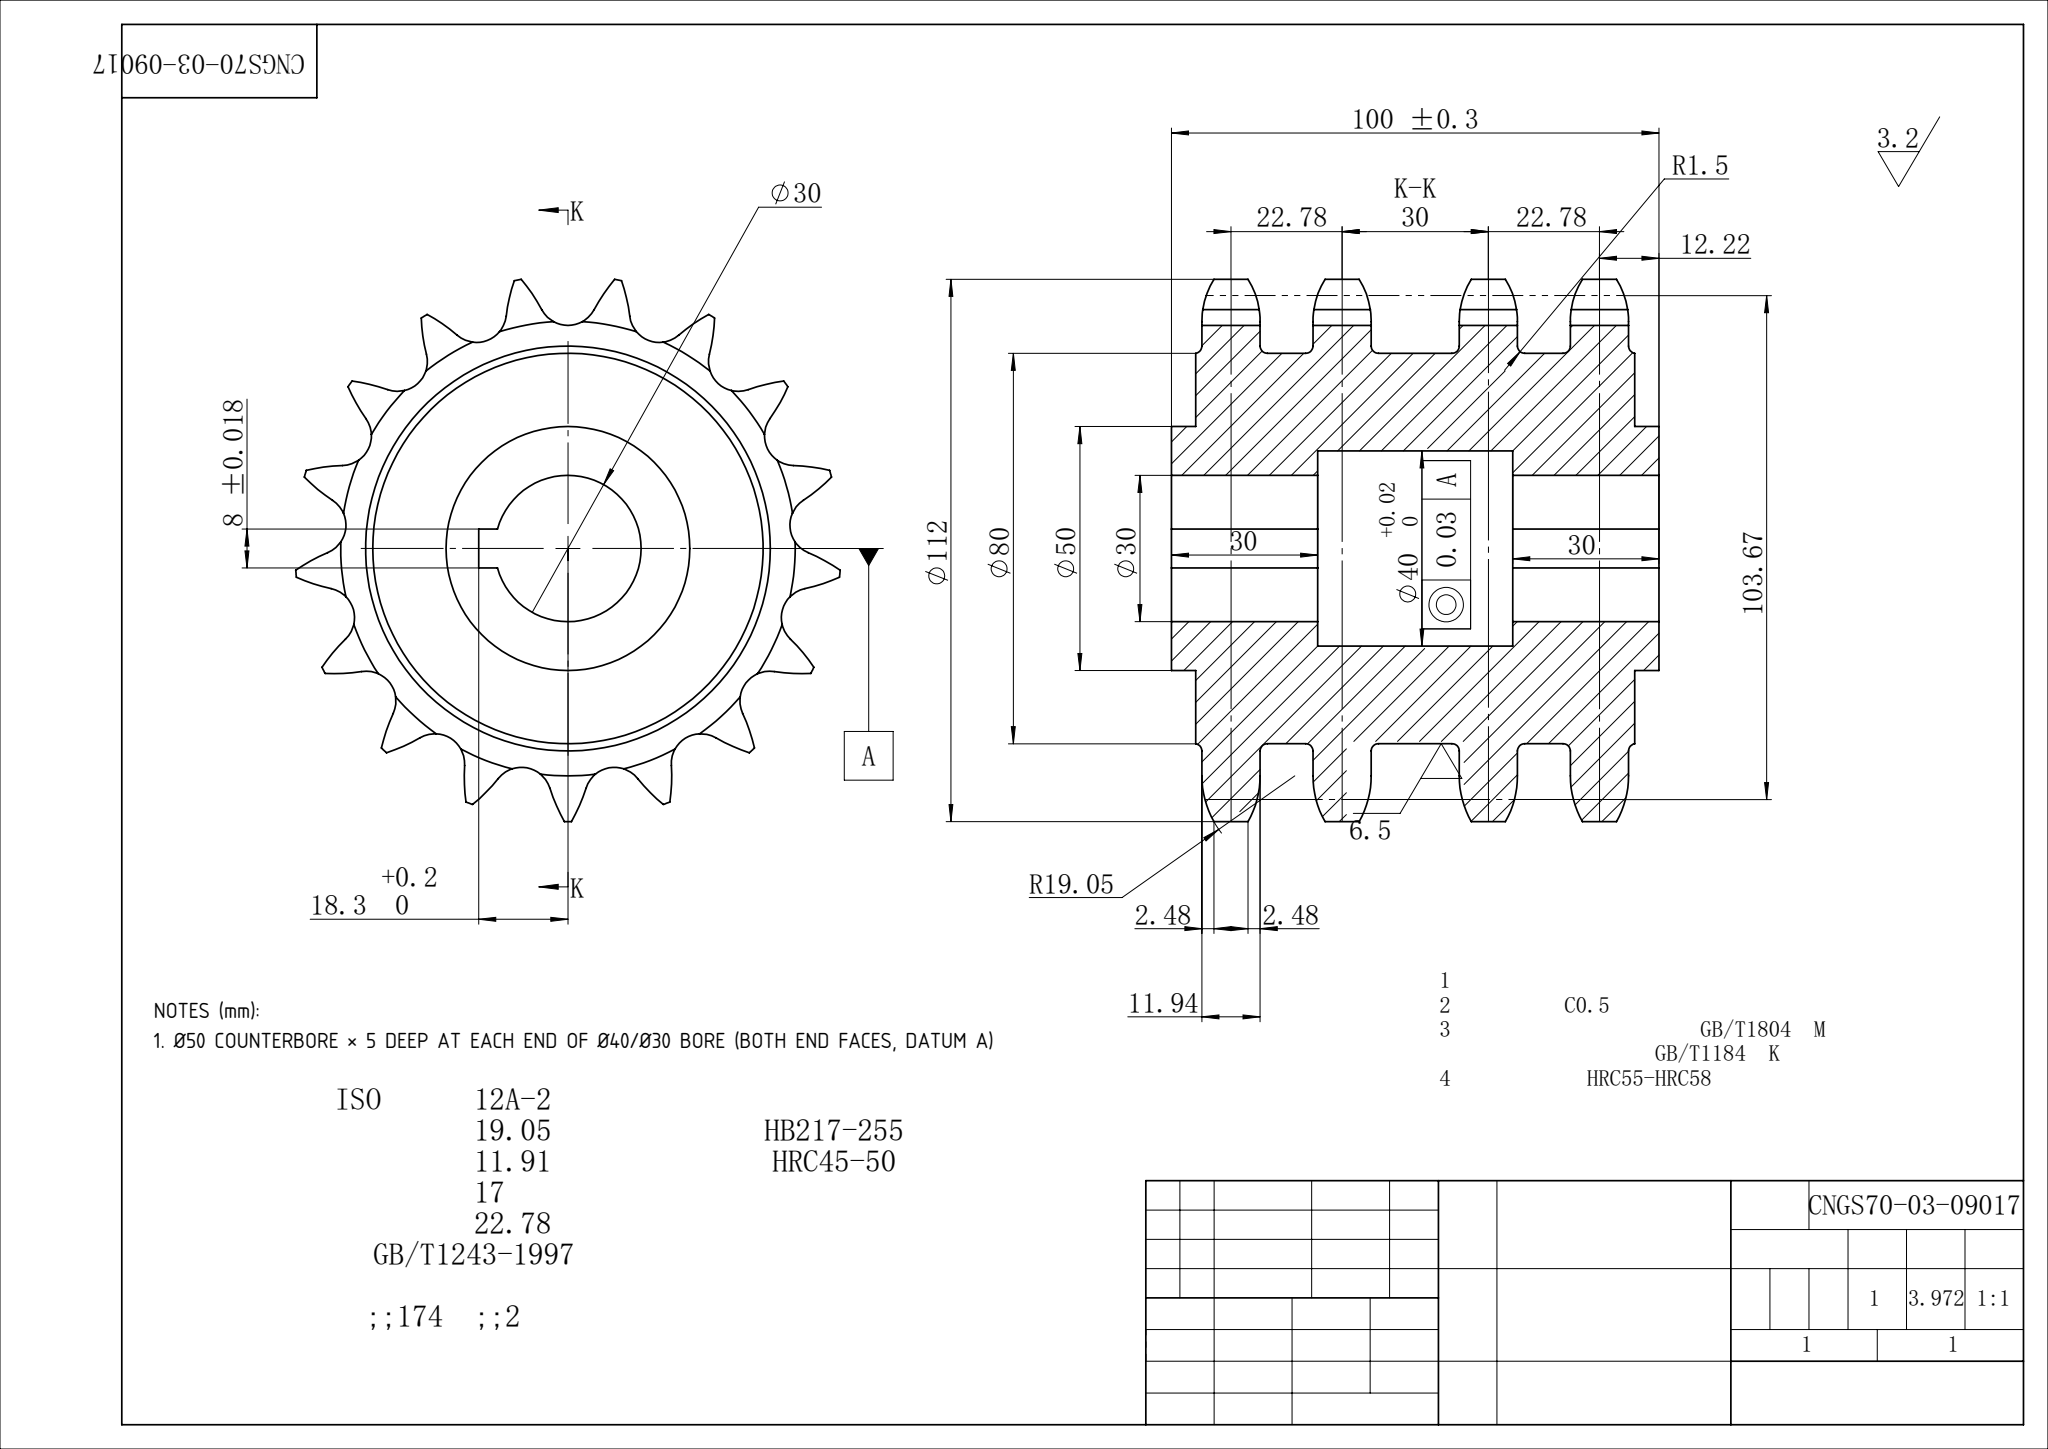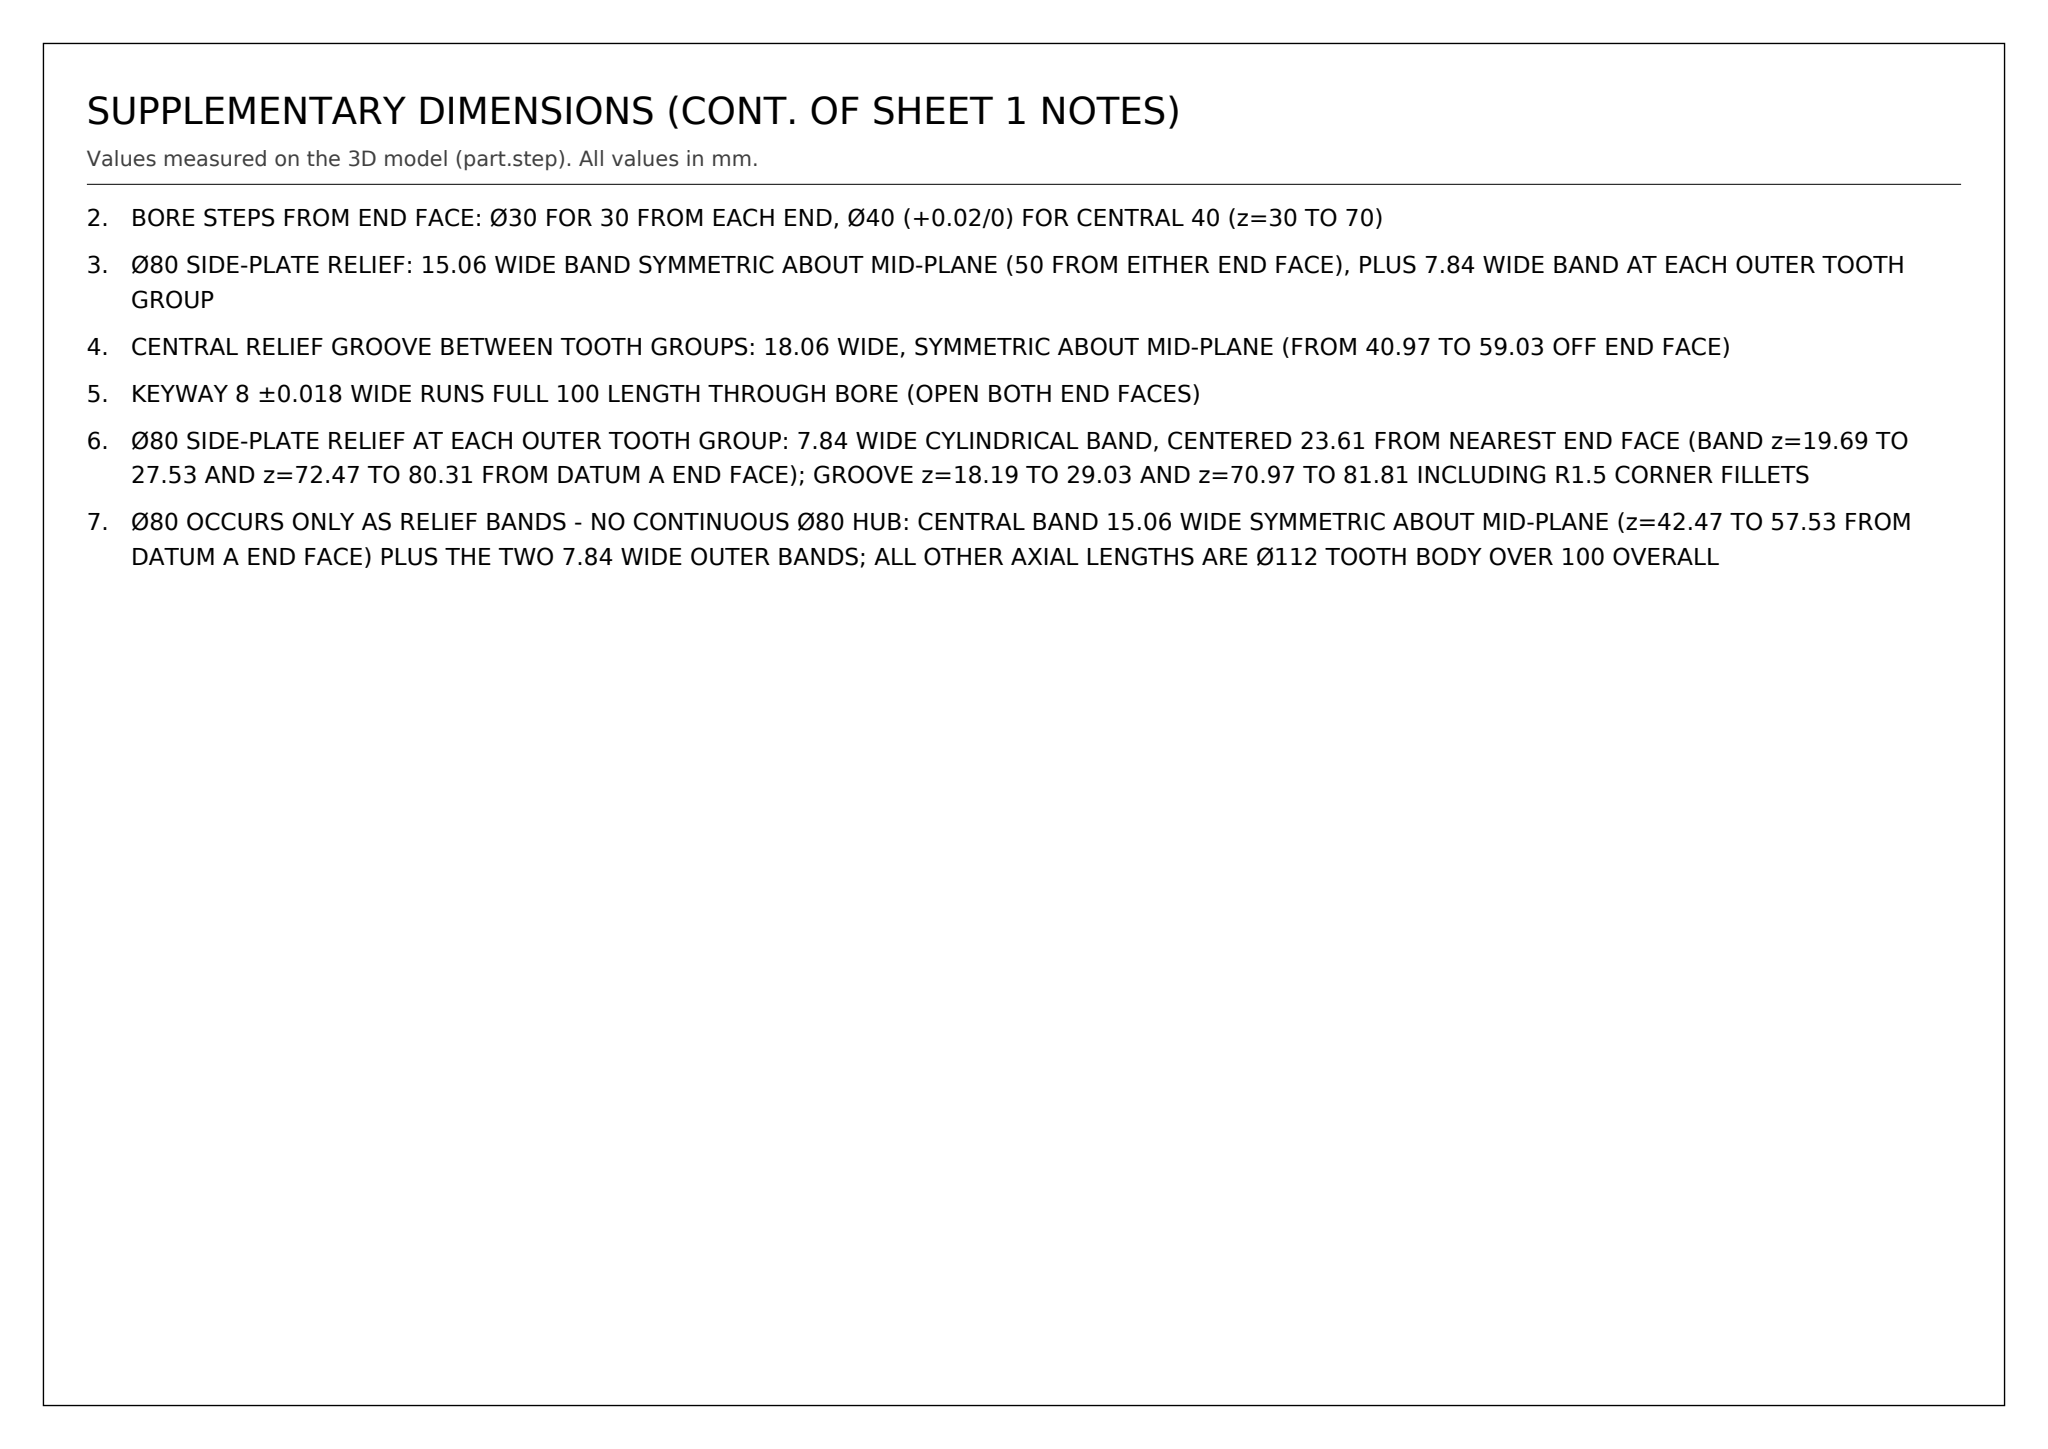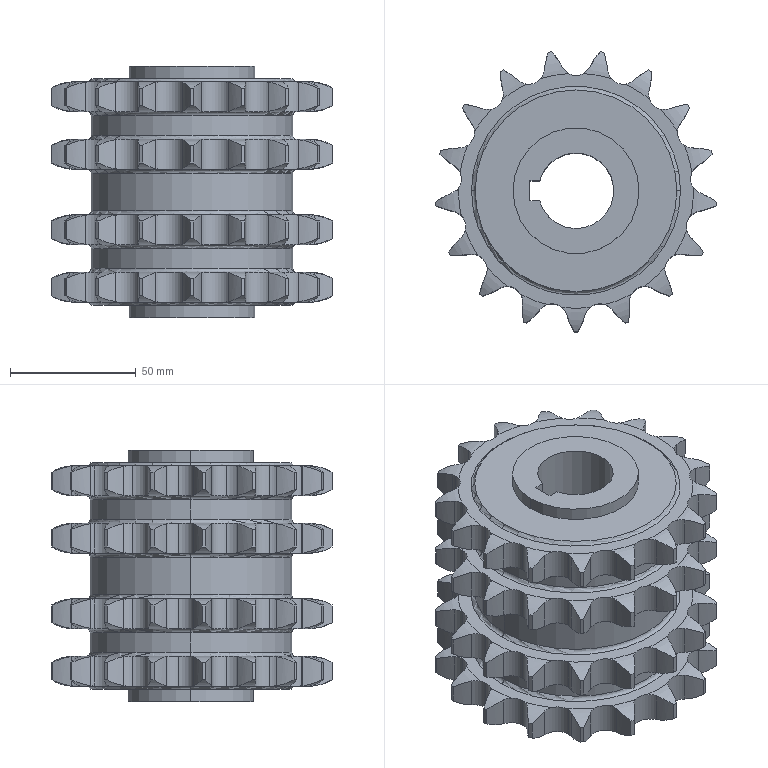Part | SolidWorks | mm | 1 solid | 494 faces | box 111.64 x 111.17 x 100 mm | volume 502766 mm3 | cylinder 314 | torus 160 | plane 20 | commonest cylinder face diameters 70 x140 12.2 x92 112 x68 80 x6 50 x4 40 x2 30 x2
Drawing notes:
Ø50 COUNTERBORE × 5 DEEP AT EACH END OF Ø40/Ø30 BORE (BOTH END FACES, DATUM A) | from the solid: cylinders: Ø50, axis z, length 5.0 (×4 faces); axis planes z=0.0/5.0 and z=95.0/100.0
BORE STEPS FROM END FACE: Ø30 FOR 30 FROM EACH END, Ø40 (+0.02/0) FOR CENTRAL 40 (z=30 TO 70) | from the solid: cylinders Ø30 L=30 (×2) and Ø40 L=40 (×2) on common axis; axis planes z=30.0 and 70.0
Ø80 SIDE-PLATE RELIEF: 15.06 WIDE BAND SYMMETRIC ABOUT MID-PLANE (50 FROM EITHER END FACE), PLUS 7.84 WIDE BAND AT EACH OUTER TOOTH GROUP | from the solid: cylinders Ø80 axis z, length 15.06 (×2 faces) and length 7.84 (×4 faces)
CENTRAL RELIEF GROOVE BETWEEN TOOTH GROUPS: 18.06 WIDE, SYMMETRIC ABOUT MID-PLANE (FROM 40.97 TO 59.03 OFF END FACE) | from the solid: axis_planes normal z at offsets 40.97 and 59.03
KEYWAY 8 ±0.018 WIDE RUNS FULL 100 LENGTH THROUGH BORE (OPEN BOTH END FACES) | from the solid: axis_planes normal y at 56.57 and 64.57 (8 apart, 2 faces only); bbox z = 100.0
Ø80 SIDE-PLATE RELIEF AT EACH OUTER TOOTH GROUP: 7.84 WIDE CYLINDRICAL BAND, CENTERED 23.61 FROM NEAREST END FACE (BAND z=19.69 TO 27.53 AND z=72.47 TO 80.31 FROM DATUM A END FACE); GROOVE z=18.19 TO 29.03 AND z=70.97 TO 81.81 INCLUDING R1.5 CORNER FILLETS | from the solid: cylinders dia 80, axis z, length 7.84 (count 4); axis_planes z = 18.19, 29.03, 70.97, 81.81; fillet_radii 1.5
Ø80 OCCURS ONLY AS RELIEF BANDS - NO CONTINUOUS Ø80 HUB: CENTRAL BAND 15.06 WIDE SYMMETRIC ABOUT MID-PLANE (z=42.47 TO 57.53 FROM DATUM A END FACE) PLUS THE TWO 7.84 WIDE OUTER BANDS; ALL OTHER AXIAL LENGTHS ARE Ø112 TOOTH BODY OVER 100 OVERALL | from the solid: cylinders dia 80 length 15.06 (count 2) and 7.84 (count 4); cylinders dia 112 length 6.98; bbox_xyz z = 100.0; axis_planes z = 40.97, 59.03, 0.0, 100.0